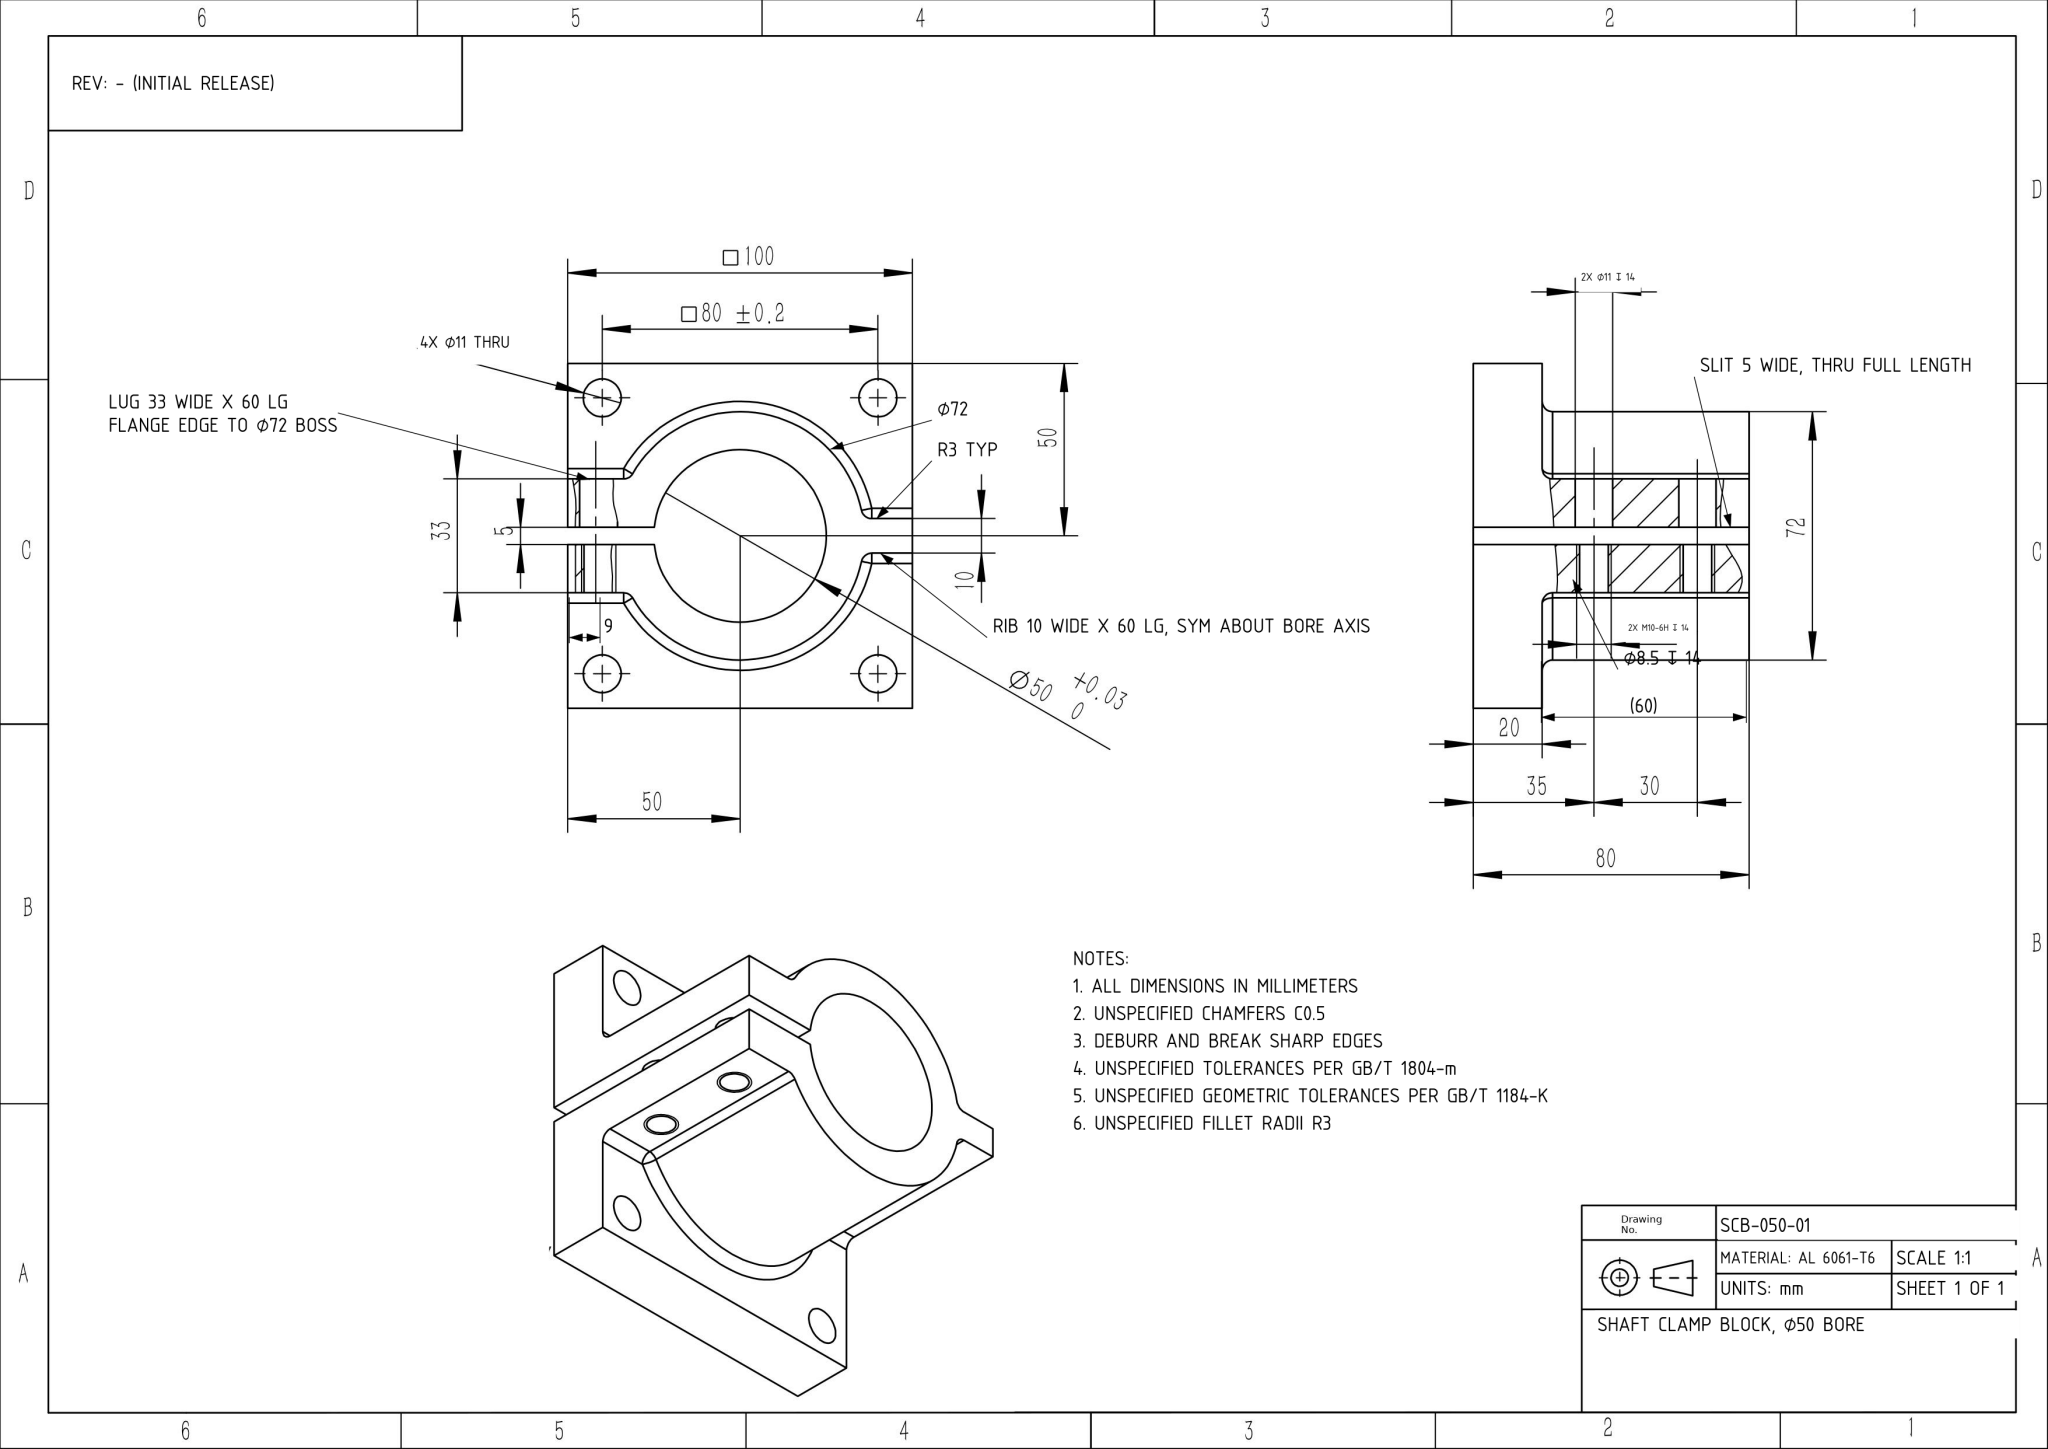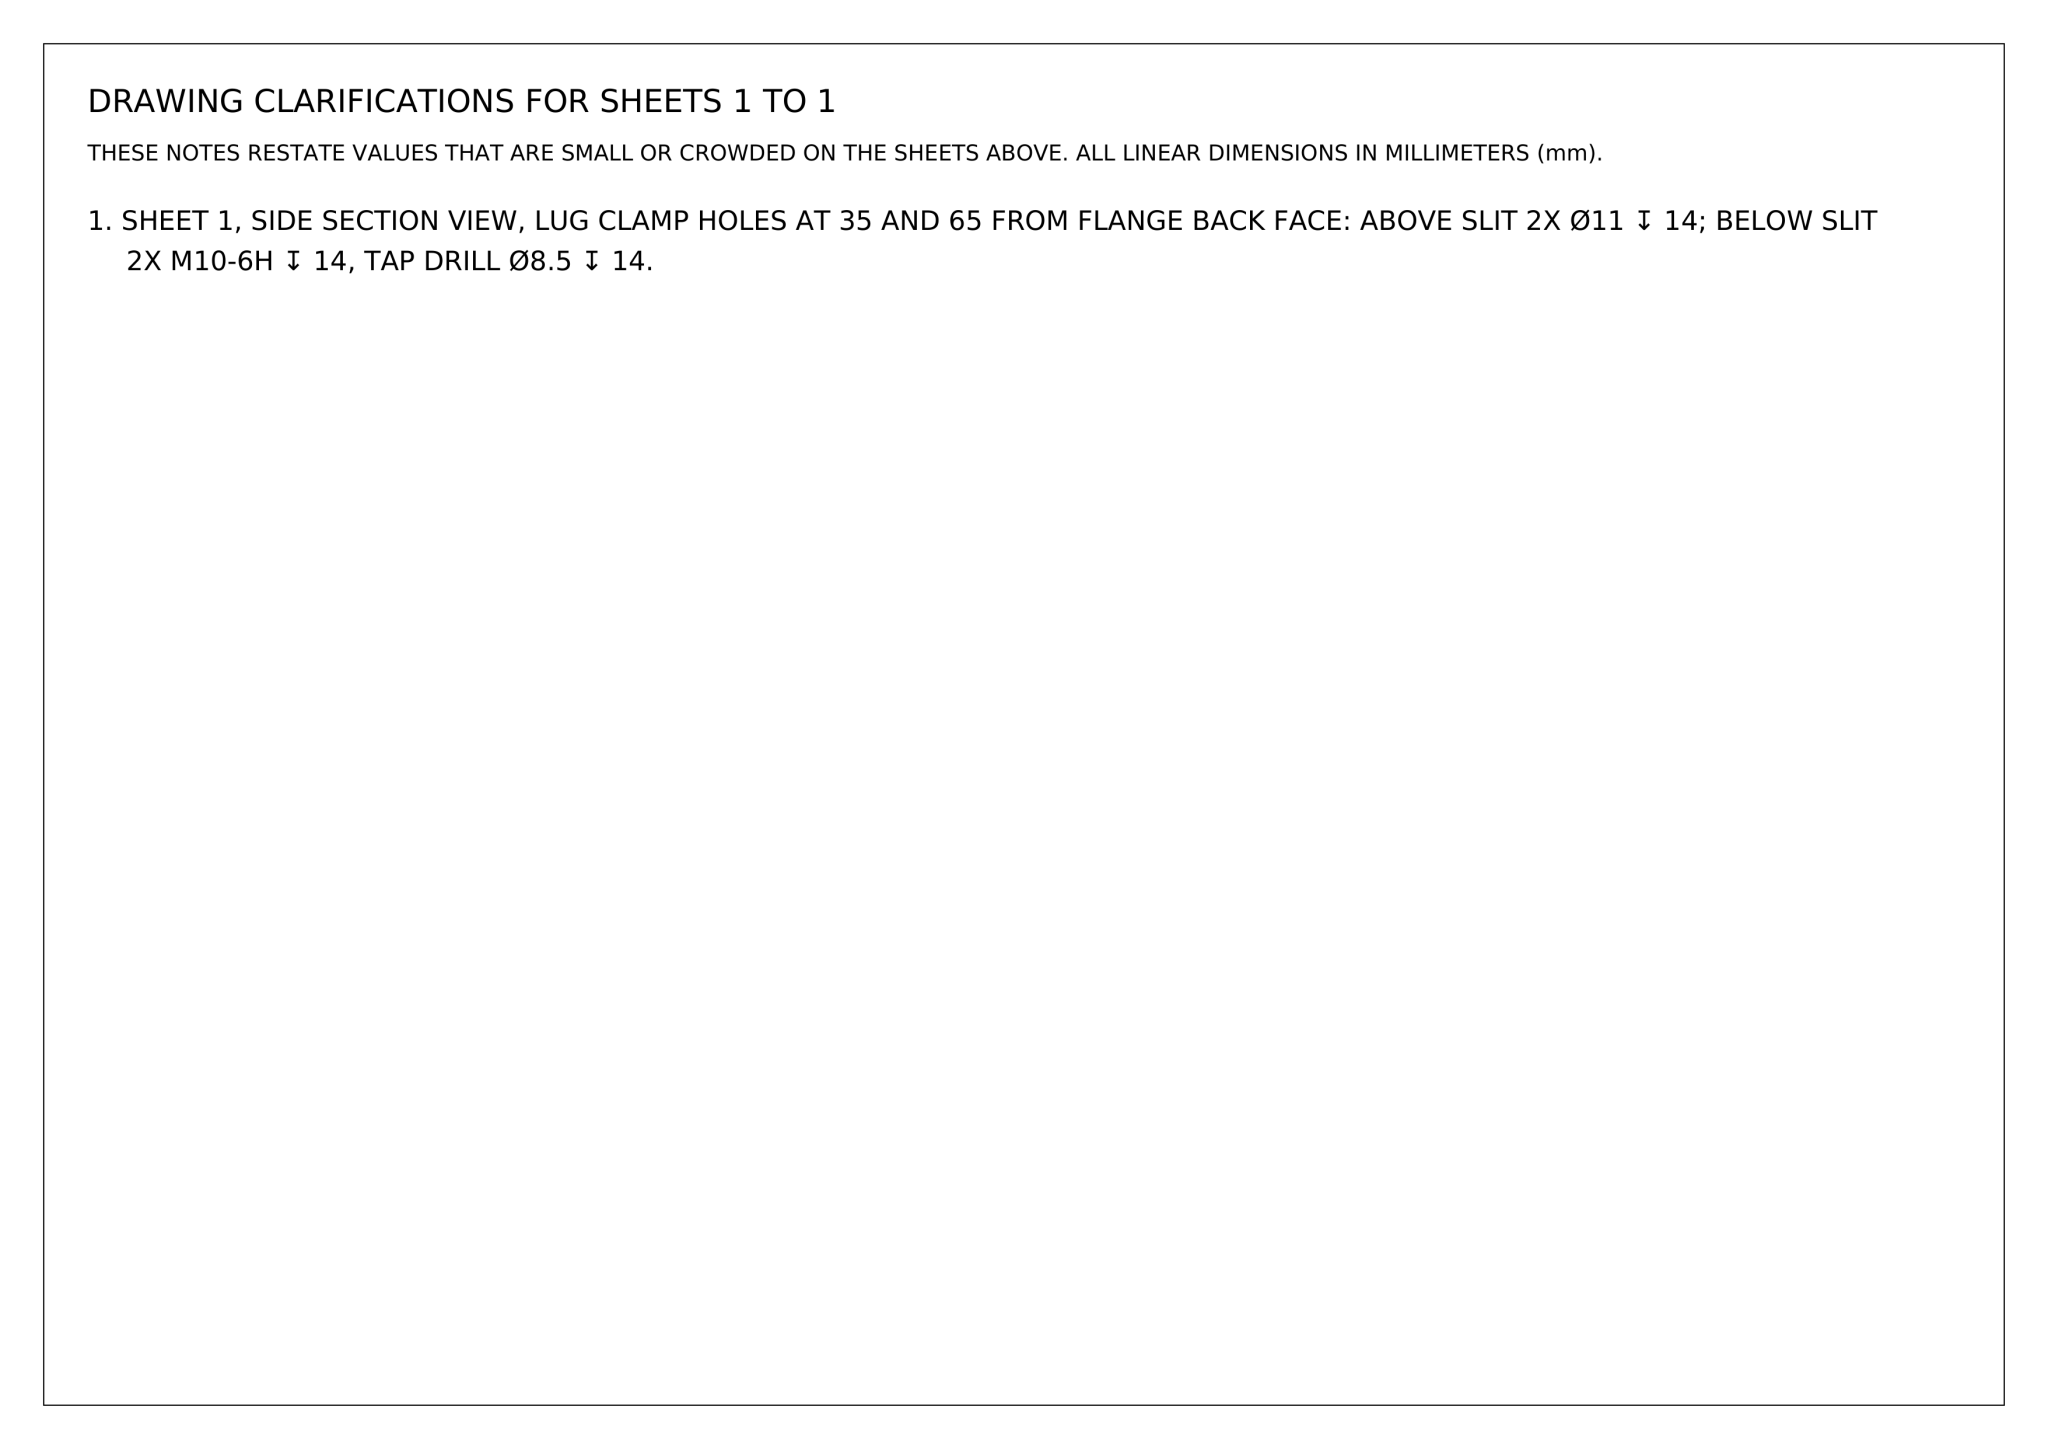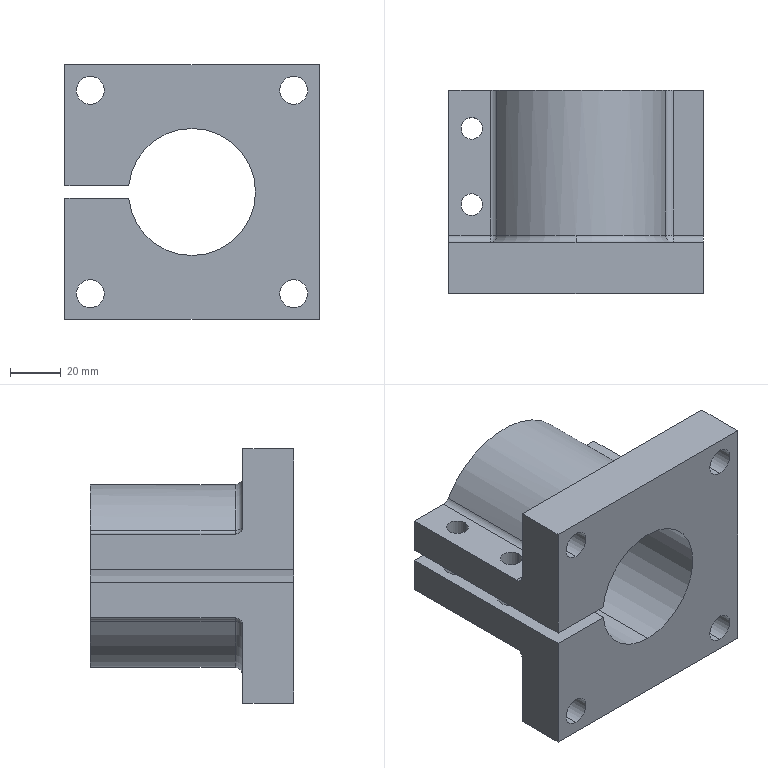Part | NX | mm | 1 solid | 52 faces | box 100 x 80 x 100 mm | volume 304793 mm3 | cylinder 30 | plane 15 | sphere 4 | torus 3 | commonest cylinder face diameters 11 x12 6 x8 8.5 x4 50 x3 72 x3